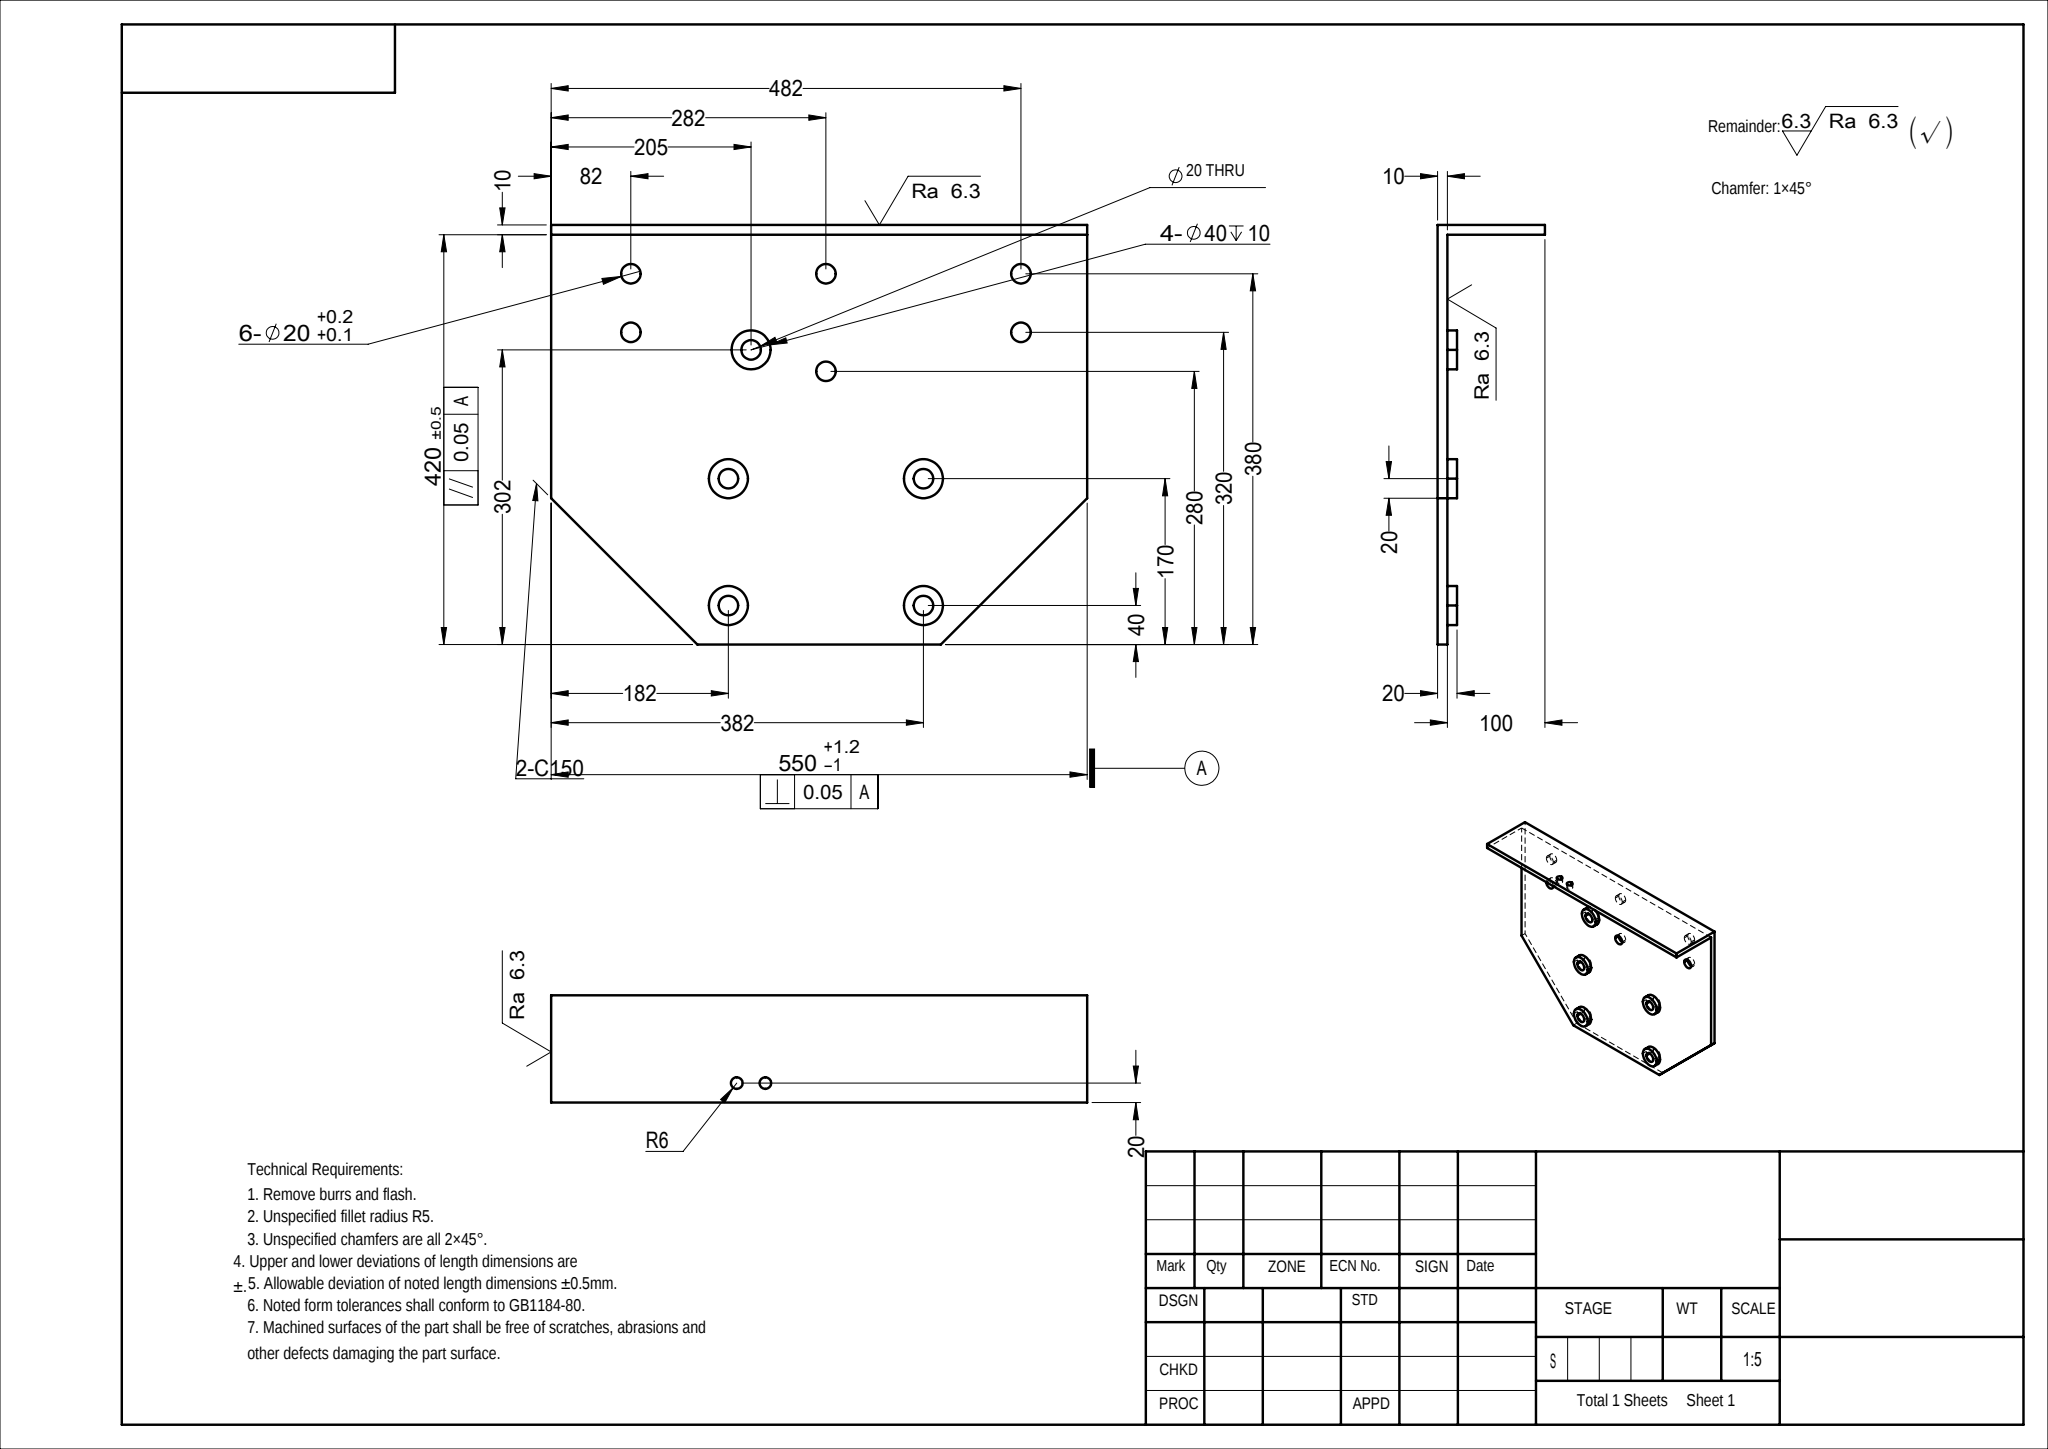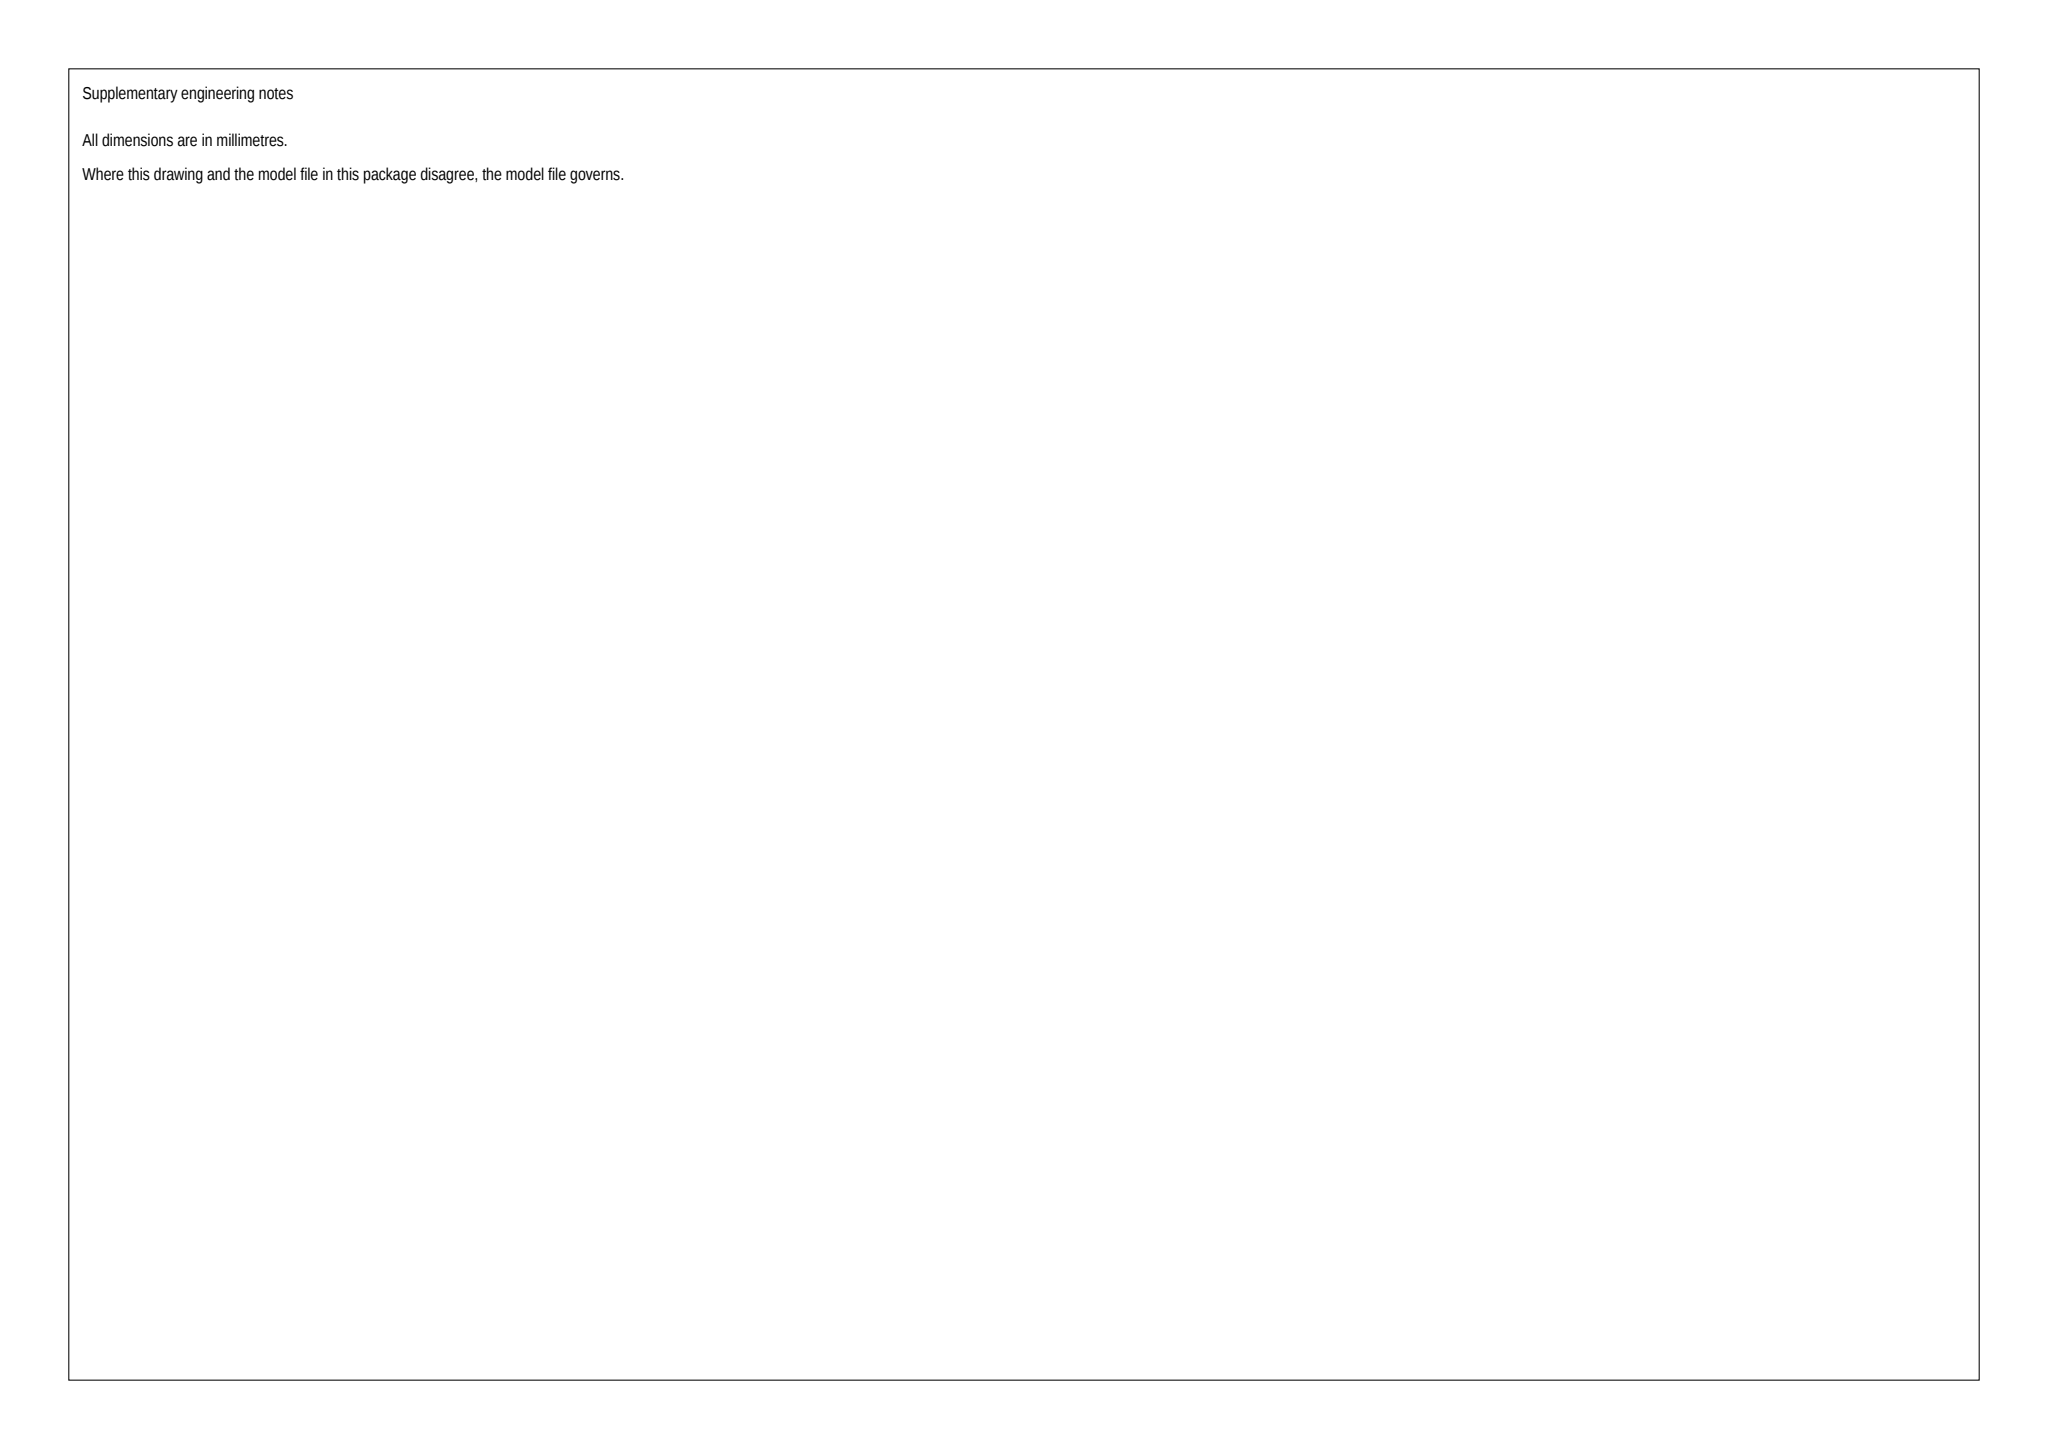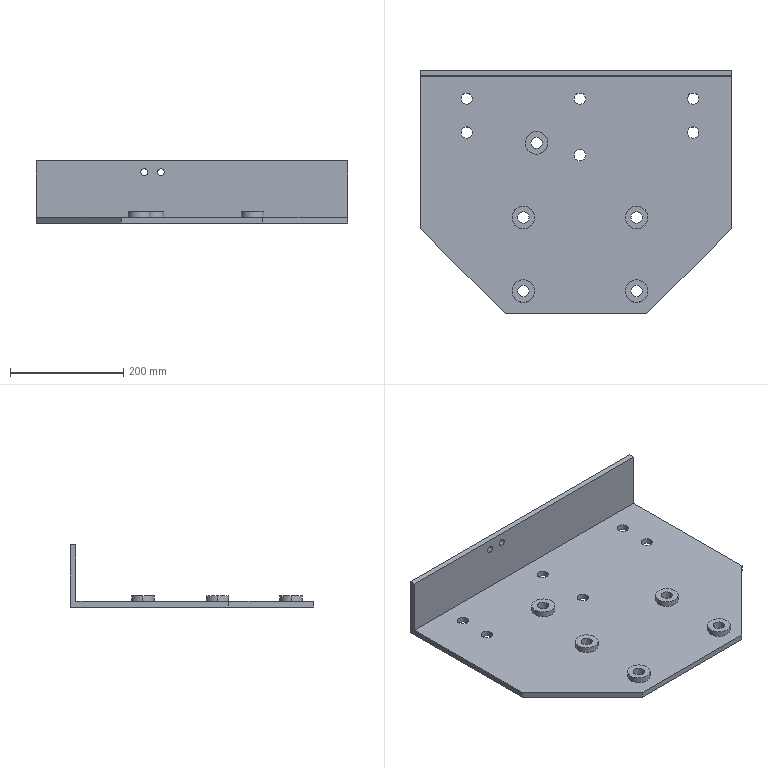Part | SolidWorks | mm | 1 solid | 51 faces | box 549.56 x 430 x 110 mm | volume 2697981 mm3 | cylinder 36 | plane 15 | commonest cylinder face diameters 20 x22 40 x10 12 x4